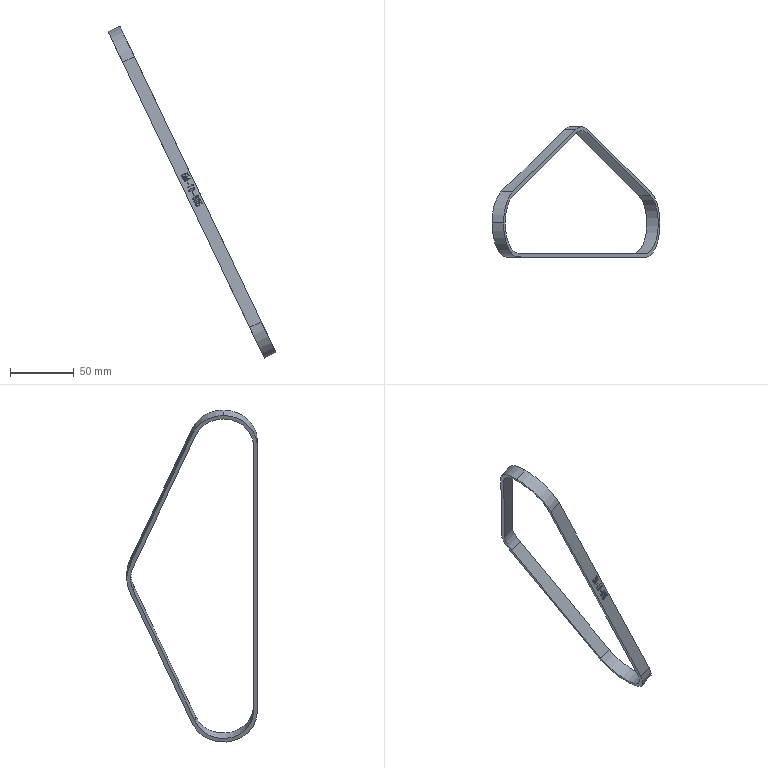Component | SolidWorks | TimingBelt5M-10-625-1 | 1 solid | 183 faces | box 131.26 x 102.19 x 259.67 mm | volume 19104 mm3 | plane 102 | spline 73 | cylinder 8 | commonest cylinder face diameters 47.1 x3 53.1 x3 56.254 x1 50.254 x1
build123d program:
from build123d import *

# Parameters (mm, degrees)
BOSS_EXTRUDE1_DEPTH = 10
SKETCH2_W           = 3.401
SKETCH2_H           = 0.341
CUT_EXTRUDE1_DEPTH  = 1


with BuildPart() as part:
    # Sketch1 → Boss-Extrude1 (new body)
    with BuildSketch(Plane.XY):
        with BuildLine():
            Line((-125.448, 13.156), (-11.068, 62.116))
            ThreePointArc((-11.068, 62.116), (0, 64.386), (11.068, 62.116))
            Line((11.068, 62.116), (125.448, 13.156))
            ThreePointArc((125.448, 13.156), (141.009, -16.584), (115, -37.802))
            Line((115, -37.802), (-115, -37.802))
            ThreePointArc((-115, -37.802), (-141.009, -16.584), (-125.448, 13.156))
        make_face()
        with BuildLine():
            Line((-124.267, 10.398), (-9.888, 59.359))
            ThreePointArc((-9.888, 59.359), (0, 61.386), (9.888, 59.359))
            Line((9.888, 59.359), (124.267, 10.398))
            ThreePointArc((124.267, 10.398), (138.07, -15.982), (115, -34.802))
            Line((115, -34.802), (-115, -34.802))
            ThreePointArc((-115, -34.802), (-138.07, -15.982), (-124.267, 10.398))
        make_face(mode=Mode.SUBTRACT)
    extrude(amount=BOSS_EXTRUDE1_DEPTH)

    # Sketch2 → Cut-Extrude1 (cut)
    # profile 1 of 9: a face of its own
    with BuildSketch(Plane.XZ.offset(37.802)):
        with BuildLine():
            add(Edge.make_bspline(
                [(-15.016, 8.016), (-14.998, 8.018), (-14.966, 8.021), (-14.934, 8.028), (-14.921, 8.031)],
                knots=[0, 0, 0, 0, 1.154, 2, 2, 2, 2], degree=3))
            Line((-14.921, 8.031), (-14.755, 8.039))
            Line((-14.755, 8.039), (-14.446, 8.086))
            Line((-14.446, 8.086), (-14.185, 8.118))
            add(Edge.make_bspline(
                [(-14.185, 8.118), (-14.161, 8.121), (-14.109, 8.13), (-14.061, 8.148), (-14.035, 8.157)],
                knots=[0, 0, 0, 0, 0.9516, 2, 2, 2, 2], degree=3))
            Line((-14.035, 8.157), (-13.917, 8.205))
            add(Edge.make_bspline(
                [(-13.917, 8.205), (-13.905, 8.21), (-13.883, 8.218), (-13.856, 8.23), (-13.836, 8.238), (-13.826, 8.243), (-13.822, 8.244)],
                knots=[0, 0, 0, 0, 1.52, 2.667, 3.508, 4, 4, 4, 4], degree=3))
            Line((-13.822, 8.244), (-13.75, 8.292))
            Line((-13.75, 8.292), (-13.521, 8.062))
            add(Edge.make_bspline(
                [(-13.521, 8.062), (-13.512, 8.051), (-13.497, 8.031), (-13.491, 7.996), (-13.499, 7.971), (-13.507, 7.949), (-13.531, 7.936), (-13.549, 7.936), (-13.56, 7.936)],
                knots=[0, 0, 0, 0, 1.453, 2.543, 3.406, 4.121, 4.875, 6, 6, 6, 6], degree=3))
            Line((-13.56, 7.936), (-15.032, 7.731))
            Line((-15.032, 7.731), (-15.056, 6.124))
            add(Edge.make_bspline(
                [(-15.056, 6.124), (-15.026, 6.16), (-14.971, 6.228), (-14.889, 6.324), (-14.793, 6.406), (-14.695, 6.458), (-14.603, 6.496), (-14.522, 6.515), (-14.432, 6.527), (-14.369, 6.528), (-14.336, 6.528)],
                knots=[0, 0, 0, 0, 1.309, 2.415, 3.508, 4.775, 5.486, 6.257, 7.088, 8, 8, 8, 8], degree=3))
            add(Edge.make_bspline(
                [(-14.336, 6.528), (-14.304, 6.526), (-14.242, 6.522), (-14.157, 6.507), (-14.082, 6.486), (-13.998, 6.442), (-13.898, 6.367), (-13.805, 6.274), (-13.732, 6.184), (-13.678, 6.108), (-13.634, 6.019), (-13.591, 5.925), (-13.553, 5.821), (-13.522, 5.707), (-13.497, 5.582), (-13.47, 5.4), (-13.447, 5.152), (-13.444, 4.949), (-13.442, 4.843)],
                knots=[0, 0, 0, 0, 0.7379, 1.395, 1.969, 2.484, 3.549, 4.783, 5.457, 6.164, 6.905, 7.691, 8.52, 9.412, 10.371, 11.392, 13.598, 16, 16, 16, 16], degree=3))
            add(Edge.make_bspline(
                [(-13.442, 4.843), (-13.444, 4.796), (-13.448, 4.704), (-13.454, 4.572), (-13.465, 4.449), (-13.481, 4.301), (-13.507, 4.131), (-13.553, 3.943), (-13.615, 3.77), (-13.699, 3.614), (-13.793, 3.478), (-13.894, 3.369), (-13.999, 3.29), (-14.11, 3.24), (-14.231, 3.217), (-14.315, 3.214), (-14.36, 3.213)],
                knots=[0, 0, 0, 0, 0.9535, 1.844, 2.674, 3.443, 4.846, 6.127, 7.335, 8.547, 9.683, 10.669, 11.53, 12.306, 13.101, 14, 14, 14, 14], degree=3))
            add(Edge.make_bspline(
                [(-14.36, 3.213), (-14.413, 3.212), (-14.513, 3.21), (-14.655, 3.227), (-14.785, 3.274), (-14.908, 3.346), (-15.023, 3.446), (-15.122, 3.57), (-15.201, 3.703), (-15.258, 3.843), (-15.293, 3.993), (-15.323, 4.157), (-15.343, 4.33), (-15.341, 4.447), (-15.341, 4.503)],
                knots=[0, 0, 0, 0, 1.038, 1.926, 2.77, 3.69, 4.673, 5.718, 6.748, 7.672, 8.626, 9.735, 10.901, 12, 12, 12, 12], degree=3))
            Line((-15.341, 4.503), (-15.332, 4.725))
            Line((-15.332, 4.725), (-15.246, 4.725))
            add(Edge.make_bspline(
                [(-15.246, 4.725), (-15.242, 4.681), (-15.235, 4.593), (-15.219, 4.462), (-15.193, 4.329), (-15.161, 4.195), (-15.12, 4.068), (-15.076, 3.951), (-15.012, 3.845), (-14.935, 3.738), (-14.836, 3.64), (-14.737, 3.572), (-14.647, 3.533), (-14.57, 3.512), (-14.483, 3.501), (-14.423, 3.499), (-14.391, 3.498)],
                knots=[0, 0, 0, 0, 1.118, 2.211, 3.325, 4.532, 5.692, 6.691, 7.681, 8.808, 10, 11.187, 11.809, 12.474, 13.201, 14, 14, 14, 14], degree=3))
            add(Edge.make_bspline(
                [(-14.391, 3.498), (-14.354, 3.498), (-14.279, 3.498), (-14.185, 3.521), (-14.11, 3.556), (-14.053, 3.597), (-13.993, 3.65), (-13.935, 3.717), (-13.878, 3.791), (-13.828, 3.872), (-13.788, 3.96), (-13.746, 4.086), (-13.707, 4.256), (-13.671, 4.476), (-13.653, 4.717), (-13.654, 4.883), (-13.655, 4.97)],
                knots=[0, 0, 0, 0, 0.8494, 1.714, 2.189, 2.722, 3.33, 4.013, 4.74, 5.462, 6.189, 6.935, 8.497, 10.189, 12.026, 14, 14, 14, 14], degree=3))
            add(Edge.make_bspline(
                [(-13.655, 4.97), (-13.658, 5.02), (-13.663, 5.116), (-13.678, 5.254), (-13.693, 5.378), (-13.72, 5.522), (-13.763, 5.688), (-13.824, 5.841), (-13.884, 5.952), (-13.933, 6.026), (-13.989, 6.088), (-14.05, 6.141), (-14.116, 6.184), (-14.185, 6.216), (-14.259, 6.237), (-14.31, 6.241), (-14.336, 6.244)],
                knots=[0, 0, 0, 0, 1.343, 2.566, 3.677, 4.66, 6.478, 8.217, 9.045, 9.823, 10.56, 11.274, 11.966, 12.641, 13.309, 14, 14, 14, 14], degree=3))
            add(Edge.make_bspline(
                [(-14.336, 6.244), (-14.364, 6.243), (-14.419, 6.241), (-14.499, 6.227), (-14.573, 6.202), (-14.661, 6.159), (-14.758, 6.094), (-14.853, 6.007), (-14.926, 5.917), (-14.96, 5.854), (-14.976, 5.824)],
                knots=[0, 0, 0, 0, 0.8403, 1.634, 2.407, 3.158, 4.57, 5.857, 6.993, 8, 8, 8, 8], degree=3))
            Line((-14.976, 5.824), (-15.032, 5.713))
            Line((-15.032, 5.713), (-15.048, 5.611))
            add(Edge.make_bspline(
                [(-15.048, 5.611), (-15.049, 5.597), (-15.05, 5.572), (-15.055, 5.539), (-15.059, 5.519), (-15.061, 5.501), (-15.08, 5.503), (-15.097, 5.52), (-15.128, 5.545), (-15.152, 5.566), (-15.166, 5.579)],
                knots=[0, 0, 0, 0, 1.417, 2.488, 3.243, 3.666, 3.979, 4.774, 6.11, 8, 8, 8, 8], degree=3))
            Line((-15.166, 5.579), (-15.332, 5.713))
            add(Edge.make_bspline(
                [(-15.332, 5.713), (-15.347, 5.726), (-15.369, 5.746), (-15.393, 5.784), (-15.375, 5.824), (-15.359, 5.849), (-15.349, 5.864)],
                knots=[0, 0, 0, 0, 1.303, 2.023, 2.754, 4, 4, 4, 4], degree=3))
            Line((-15.349, 5.864), (-15.261, 5.982))
            Line((-15.261, 5.982), (-15.246, 6.828))
            Line((-15.246, 6.828), (-15.238, 7.438))
            add(Edge.make_bspline(
                [(-15.238, 7.438), (-15.238, 7.46), (-15.238, 7.509), (-15.238, 7.587), (-15.237, 7.675), (-15.238, 7.768), (-15.237, 7.858), (-15.24, 7.934), (-15.241, 7.993), (-15.244, 8.025), (-15.246, 8.039)],
                knots=[0, 0, 0, 0, 0.9041, 1.949, 3.118, 4.412, 5.659, 6.688, 7.452, 8, 8, 8, 8], degree=3))
            Line((-15.246, 8.039), (-15.277, 8.284))
            Line((-15.277, 8.284), (-15.198, 8.316))
            add(Edge.make_bspline(
                [(-15.198, 8.316), (-15.186, 8.286), (-15.167, 8.237), (-15.139, 8.171), (-15.105, 8.122), (-15.078, 8.094), (-15.064, 8.079)],
                knots=[0, 0, 0, 0, 1.379, 2.319, 3.105, 4, 4, 4, 4], degree=3))
            Line((-15.064, 8.079), (-15.016, 8.016))
        make_face()
    # profile 2 of 9: a face of its own
    with BuildSketch(Plane.XZ.offset(37.802)):
        with BuildLine():
            Line((-10.449, 8.347), (-10.267, 8.347))
            Line((-10.267, 8.347), (-10.157, 4.637))
            Line((-10.157, 4.637), (-10.149, 4.289))
            add(Edge.make_bspline(
                [(-10.149, 4.289), (-10.148, 4.25), (-10.148, 4.184), (-10.142, 4.096), (-10.13, 4.023), (-10.115, 3.953), (-10.094, 3.886), (-10.073, 3.829), (-10.052, 3.788), (-10.04, 3.755), (-10.046, 3.723), (-10.055, 3.683), (-10.076, 3.625), (-10.092, 3.58), (-10.101, 3.554)],
                knots=[0, 0, 0, 0, 1.834, 3.115, 4.183, 5.36, 6.502, 7.475, 8.229, 8.746, 9.081, 9.728, 10.706, 12, 12, 12, 12], degree=3))
            Line((-10.101, 3.554), (-10.189, 3.284))
            add(Edge.make_bspline(
                [(-10.189, 3.284), (-10.198, 3.26), (-10.215, 3.216), (-10.239, 3.16), (-10.255, 3.122), (-10.271, 3.097), (-10.287, 3.084), (-10.307, 3.08), (-10.322, 3.093), (-10.328, 3.104), (-10.331, 3.111)],
                knots=[0, 0, 0, 0, 2.257, 3.989, 5.166, 5.812, 6.432, 6.936, 7.389, 8, 8, 8, 8], degree=3))
            add(Edge.make_bspline(
                [(-10.331, 3.111), (-10.335, 3.121), (-10.348, 3.145), (-10.348, 3.196), (-10.348, 3.265), (-10.342, 3.318), (-10.339, 3.348)],
                knots=[0, 0, 0, 0, 0.5334, 1.357, 2.51, 4, 4, 4, 4], degree=3))
            Line((-10.339, 3.348), (-10.354, 3.846))
            Line((-10.354, 3.846), (-10.449, 7.271))
            Line((-10.449, 7.271), (-11.335, 3.253))
            Line((-11.335, 3.253), (-11.486, 3.261))
            Line((-11.486, 3.261), (-12.442, 7.225))
            Line((-12.442, 7.225), (-12.506, 3.807))
            Line((-12.506, 3.807), (-12.522, 3.316))
            add(Edge.make_bspline(
                [(-12.522, 3.316), (-12.522, 3.28), (-12.523, 3.217), (-12.534, 3.143), (-12.545, 3.098), (-12.554, 3.077), (-12.564, 3.062), (-12.573, 3.063), (-12.577, 3.063)],
                knots=[0, 0, 0, 0, 2.359, 4.22, 4.917, 5.428, 5.74, 6, 6, 6, 6], degree=3))
            add(Edge.make_bspline(
                [(-12.577, 3.063), (-12.583, 3.064), (-12.594, 3.066), (-12.616, 3.076), (-12.632, 3.112), (-12.646, 3.153), (-12.659, 3.192), (-12.665, 3.217), (-12.671, 3.233), (-12.672, 3.242), (-12.672, 3.245)],
                knots=[0, 0, 0, 0, 0.6183, 1.294, 2.516, 4.811, 6.123, 7.066, 7.695, 8, 8, 8, 8], degree=3))
            Line((-12.672, 3.245), (-12.815, 3.601))
            add(Edge.make_bspline(
                [(-12.815, 3.601), (-12.819, 3.619), (-12.827, 3.654), (-12.825, 3.709), (-12.81, 3.768), (-12.788, 3.829), (-12.765, 3.885), (-12.749, 3.927), (-12.74, 3.958), (-12.736, 3.99), (-12.731, 4.031), (-12.728, 4.079), (-12.725, 4.128), (-12.721, 4.17), (-12.72, 4.201), (-12.717, 4.223), (-12.715, 4.241), (-12.714, 4.264), (-12.713, 4.296), (-12.71, 4.338), (-12.71, 4.389), (-12.707, 4.45), (-12.706, 4.521), (-12.705, 4.571), (-12.704, 4.598)],
                knots=[0, 0, 0, 0, 1.188, 2.333, 3.586, 5.123, 6.574, 7.524, 7.999, 8.693, 9.59, 10.712, 11.859, 12.753, 13.442, 13.903, 14.184, 14.668, 15.356, 16.273, 17.393, 18.717, 20.244, 22, 22, 22, 22], degree=3))
            Line((-12.704, 4.598), (-12.649, 8.347))
            Line((-12.649, 8.347), (-12.459, 8.347))
            Line((-12.459, 8.347), (-11.423, 3.87))
            Line((-11.423, 3.87), (-10.449, 8.347))
        make_face()
    # profile 3 of 9: a face of its own
    with BuildSketch(Plane.XZ.offset(37.802)):
        with Locations((-7.963, 5.155)):
            Rectangle(SKETCH2_W, SKETCH2_H)
    # profile 4 of 9: a face of its own
    with BuildSketch(Plane.XZ.offset(37.802)):
        with BuildLine():
            Line((-4.557, 8.3), (-4.471, 8.3))
            Line((-4.471, 8.3), (-4.479, 4.099))
            add(Edge.make_bspline(
                [(-4.479, 4.099), (-4.48, 4.061), (-4.482, 3.988), (-4.482, 3.884), (-4.485, 3.79), (-4.486, 3.706), (-4.488, 3.631), (-4.491, 3.566), (-4.491, 3.511), (-4.496, 3.425), (-4.503, 3.306), (-4.518, 3.184), (-4.53, 3.097), (-4.543, 3.057), (-4.558, 3.026), (-4.574, 3.03), (-4.581, 3.031)],
                knots=[0, 0, 0, 0, 1.45, 2.781, 3.977, 5.054, 6.011, 6.834, 7.536, 8.12, 10.143, 12.069, 12.873, 13.44, 13.76, 14, 14, 14, 14], degree=3))
            add(Edge.make_bspline(
                [(-4.581, 3.031), (-4.582, 3.032), (-4.589, 3.037), (-4.605, 3.048), (-4.624, 3.077), (-4.632, 3.102), (-4.637, 3.118)],
                knots=[0, 0, 0, 0, 0.2213, 0.9471, 2.151, 4, 4, 4, 4], degree=3))
            Line((-4.637, 3.118), (-4.676, 3.221))
            Line((-4.676, 3.221), (-4.764, 3.506))
            add(Edge.make_bspline(
                [(-4.764, 3.506), (-4.774, 3.533), (-4.793, 3.579), (-4.811, 3.641), (-4.825, 3.68), (-4.829, 3.712), (-4.811, 3.742), (-4.798, 3.787), (-4.777, 3.846), (-4.758, 3.915), (-4.741, 3.99), (-4.726, 4.071), (-4.717, 4.162), (-4.713, 4.248), (-4.709, 4.332), (-4.709, 4.413), (-4.707, 4.508), (-4.707, 4.577), (-4.707, 4.613)],
                knots=[0, 0, 0, 0, 1.22, 2.126, 2.712, 2.994, 3.44, 4.126, 5.031, 6.063, 7.167, 8.277, 9.542, 11.034, 11.961, 13.087, 14.444, 16, 16, 16, 16], degree=3))
            Line((-4.707, 4.613), (-4.7, 7.714))
            Line((-4.7, 7.714), (-5.112, 7.358))
            Line((-5.112, 7.358), (-5.143, 7.493))
            add(Edge.make_bspline(
                [(-5.143, 7.493), (-5.11, 7.527), (-5.047, 7.592), (-4.964, 7.685), (-4.895, 7.766), (-4.823, 7.861), (-4.743, 7.979), (-4.683, 8.075), (-4.652, 8.126)],
                knots=[0, 0, 0, 0, 1.077, 2.019, 2.808, 3.458, 4.679, 6, 6, 6, 6], degree=3))
            Line((-4.652, 8.126), (-4.557, 8.3))
        make_face()
    # profile 5 of 9: a face of its own
    with BuildSketch(Plane.XZ.offset(37.802)):
        with BuildLine():
            add(Edge.make_bspline(
                [(-2.673, 5.832), (-2.669, 5.908), (-2.661, 6.063), (-2.64, 6.301), (-2.609, 6.55), (-2.572, 6.805), (-2.522, 7.057), (-2.458, 7.297), (-2.375, 7.518), (-2.293, 7.688), (-2.224, 7.813), (-2.173, 7.896), (-2.125, 7.971), (-2.078, 8.036), (-2.032, 8.091), (-1.989, 8.139), (-1.945, 8.177), (-1.891, 8.214), (-1.825, 8.247), (-1.749, 8.276), (-1.675, 8.292), (-1.627, 8.292), (-1.604, 8.292)],
                knots=[0, 0, 0, 0, 1.583, 3.244, 4.984, 6.805, 8.617, 10.34, 11.975, 13.538, 14.275, 14.951, 15.564, 16.129, 16.627, 17.071, 17.469, 17.815, 18.438, 19.003, 19.519, 20, 20, 20, 20], degree=3))
            add(Edge.make_bspline(
                [(-1.604, 8.292), (-1.582, 8.288), (-1.535, 8.28), (-1.466, 8.25), (-1.393, 8.209), (-1.315, 8.157), (-1.237, 8.087), (-1.165, 7.993), (-1.098, 7.88), (-1.015, 7.7), (-0.9231, 7.455), (-0.8511, 7.199), (-0.8044, 6.985), (-0.7739, 6.814), (-0.7496, 6.633), (-0.7235, 6.378), (-0.7003, 6.052), (-0.6966, 5.789), (-0.6947, 5.658)],
                knots=[0, 0, 0, 0, 0.3637, 0.7682, 1.217, 1.725, 2.291, 2.915, 3.632, 4.434, 6.138, 7.867, 8.757, 9.699, 10.686, 11.727, 13.859, 16, 16, 16, 16], degree=3))
            add(Edge.make_bspline(
                [(-0.6947, 5.658), (-0.7019, 5.552), (-0.7166, 5.335), (-0.7517, 5.003), (-0.8095, 4.657), (-0.8823, 4.366), (-0.9528, 4.135), (-1.012, 3.967), (-1.079, 3.81), (-1.151, 3.662), (-1.225, 3.531), (-1.302, 3.421), (-1.383, 3.337), (-1.466, 3.276), (-1.547, 3.235), (-1.625, 3.208), (-1.699, 3.194), (-1.747, 3.196), (-1.771, 3.198)],
                knots=[0, 0, 0, 0, 1.76, 3.618, 5.557, 7.587, 8.607, 9.588, 10.541, 11.46, 12.308, 13.044, 13.688, 14.251, 14.754, 15.2, 15.616, 16, 16, 16, 16], degree=3))
            add(Edge.make_bspline(
                [(-1.771, 3.198), (-1.793, 3.201), (-1.839, 3.207), (-1.909, 3.235), (-1.982, 3.277), (-2.06, 3.333), (-2.139, 3.41), (-2.214, 3.509), (-2.287, 3.631), (-2.355, 3.774), (-2.42, 3.934), (-2.477, 4.106), (-2.529, 4.286), (-2.571, 4.475), (-2.606, 4.666), (-2.633, 4.854), (-2.652, 5.036), (-2.662, 5.212), (-2.666, 5.38), (-2.67, 5.54), (-2.672, 5.689), (-2.673, 5.786), (-2.673, 5.832)],
                knots=[0, 0, 0, 0, 0.4512, 0.9506, 1.515, 2.163, 2.892, 3.734, 4.688, 5.773, 6.954, 8.176, 9.446, 10.772, 12.102, 13.384, 14.62, 15.819, 16.962, 18.041, 19.056, 20, 20, 20, 20], degree=3))
        make_face()
        with BuildLine():
            add(Edge.make_bspline(
                [(-2.467, 5.816), (-2.468, 5.778), (-2.469, 5.697), (-2.471, 5.569), (-2.468, 5.427), (-2.462, 5.216), (-2.443, 4.941), (-2.392, 4.611), (-2.32, 4.291), (-2.241, 4.041), (-2.167, 3.862), (-2.111, 3.751), (-2.051, 3.662), (-1.989, 3.594), (-1.926, 3.545), (-1.867, 3.511), (-1.811, 3.487), (-1.773, 3.484), (-1.755, 3.482)],
                knots=[0, 0, 0, 0, 0.7057, 1.499, 2.386, 3.361, 5.418, 7.515, 9.574, 11.515, 12.399, 13.17, 13.83, 14.396, 14.883, 15.304, 15.67, 16, 16, 16, 16], degree=3))
            add(Edge.make_bspline(
                [(-1.755, 3.482), (-1.739, 3.483), (-1.704, 3.483), (-1.648, 3.496), (-1.59, 3.524), (-1.526, 3.561), (-1.459, 3.618), (-1.394, 3.695), (-1.33, 3.794), (-1.266, 3.912), (-1.205, 4.042), (-1.151, 4.18), (-1.104, 4.323), (-1.053, 4.523), (-1.001, 4.781), (-0.9537, 5.098), (-0.9225, 5.409), (-0.9095, 5.664), (-0.9059, 5.865), (-0.9089, 6.025), (-0.9146, 6.197), (-0.921, 6.316), (-0.9244, 6.377)],
                knots=[0, 0, 0, 0, 0.3081, 0.6619, 1.055, 1.515, 2.051, 2.68, 3.41, 4.262, 5.184, 6.105, 7.046, 8, 9.968, 11.998, 13.994, 15.843, 16.773, 17.77, 18.848, 20, 20, 20, 20], degree=3))
            add(Edge.make_bspline(
                [(-0.9244, 6.377), (-0.9301, 6.435), (-0.941, 6.546), (-0.9603, 6.707), (-0.9842, 6.857), (-1.018, 7.041), (-1.072, 7.262), (-1.147, 7.473), (-1.212, 7.632), (-1.268, 7.732), (-1.324, 7.818), (-1.387, 7.883), (-1.448, 7.934), (-1.506, 7.972), (-1.56, 7.999), (-1.596, 8.005), (-1.612, 8.007)],
                knots=[0, 0, 0, 0, 1.303, 2.529, 3.662, 4.721, 6.756, 8.792, 9.76, 10.624, 11.385, 12.064, 12.659, 13.175, 13.621, 14, 14, 14, 14], degree=3))
            add(Edge.make_bspline(
                [(-1.612, 8.007), (-1.63, 8.006), (-1.668, 8.003), (-1.726, 7.986), (-1.788, 7.958), (-1.856, 7.919), (-1.926, 7.857), (-1.997, 7.767), (-2.071, 7.647), (-2.147, 7.499), (-2.221, 7.324), (-2.283, 7.125), (-2.337, 6.903), (-2.378, 6.666), (-2.41, 6.429), (-2.436, 6.206), (-2.456, 6.004), (-2.463, 5.876), (-2.467, 5.816)],
                knots=[0, 0, 0, 0, 0.3474, 0.73, 1.157, 1.645, 2.22, 2.946, 3.85, 4.924, 6.146, 7.478, 8.938, 10.524, 12.101, 13.544, 14.841, 16, 16, 16, 16], degree=3))
        make_face(mode=Mode.SUBTRACT)
    # profile 6 of 9: a face of its own
    with BuildSketch(Plane.XZ.offset(37.802)):
        with Locations((1.713, 5.155)):
            Rectangle(SKETCH2_W, SKETCH2_H)
    # profile 7 of 9: a face of its own
    with BuildSketch(Plane.XZ.offset(37.802)):
        with BuildLine():
            Line((6.019, 6.797), (5.909, 6.797))
            add(Edge.make_bspline(
                [(5.909, 6.797), (5.902, 6.844), (5.887, 6.937), (5.873, 7.08), (5.856, 7.228), (5.828, 7.385), (5.783, 7.548), (5.719, 7.678), (5.659, 7.775), (5.608, 7.84), (5.549, 7.895), (5.487, 7.941), (5.419, 7.976), (5.348, 8.002), (5.273, 8.013), (5.197, 8.012), (5.122, 8.004), (5.053, 7.986), (4.991, 7.961), (4.933, 7.929), (4.88, 7.882), (4.824, 7.824), (4.769, 7.747), (4.711, 7.657), (4.654, 7.552), (4.605, 7.432), (4.56, 7.299), (4.509, 7.103), (4.461, 6.839), (4.432, 6.569), (4.418, 6.358), (4.412, 6.216), (4.406, 6.093), (4.406, 6.017), (4.406, 5.982)],
                knots=[0, 0, 0, 0, 1.173, 2.32, 3.517, 4.833, 6.232, 7.655, 8.357, 9.032, 9.677, 10.315, 10.933, 11.542, 12.153, 12.786, 13.414, 13.988, 14.535, 15.054, 15.605, 16.263, 17.03, 17.918, 18.896, 19.957, 21.1, 22.329, 24.933, 27.662, 28.978, 30.14, 31.147, 32, 32, 32, 32], degree=3))
            Line((4.406, 5.982), (4.399, 5.674))
            add(Edge.make_bspline(
                [(4.399, 5.674), (4.418, 5.729), (4.454, 5.829), (4.508, 5.967), (4.569, 6.083), (4.641, 6.191), (4.734, 6.291), (4.828, 6.364), (4.918, 6.414), (4.997, 6.443), (5.086, 6.463), (5.149, 6.469), (5.182, 6.472)],
                knots=[0, 0, 0, 0, 1.464, 2.646, 3.694, 4.755, 5.874, 7.079, 7.725, 8.423, 9.174, 10, 10, 10, 10], degree=3))
            add(Edge.make_bspline(
                [(5.182, 6.472), (5.229, 6.47), (5.319, 6.467), (5.45, 6.428), (5.571, 6.36), (5.665, 6.276), (5.741, 6.194), (5.797, 6.118), (5.851, 6.033), (5.921, 5.905), (5.996, 5.73), (6.051, 5.544), (6.079, 5.386), (6.098, 5.259), (6.107, 5.123), (6.113, 4.933), (6.11, 4.696), (6.097, 4.507), (6.091, 4.415)],
                knots=[0, 0, 0, 0, 0.9091, 1.729, 2.577, 3.565, 4.121, 4.72, 5.36, 6.06, 7.513, 8.994, 9.771, 10.587, 11.458, 12.38, 14.23, 16, 16, 16, 16], degree=3))
            add(Edge.make_bspline(
                [(6.091, 4.415), (6.084, 4.368), (6.068, 4.269), (6.036, 4.116), (5.996, 3.954), (5.95, 3.788), (5.897, 3.63), (5.827, 3.496), (5.742, 3.391), (5.645, 3.318), (5.548, 3.271), (5.461, 3.234), (5.386, 3.207), (5.338, 3.201), (5.316, 3.198)],
                knots=[0, 0, 0, 0, 1.11, 2.303, 3.588, 4.949, 6.256, 7.397, 8.411, 9.334, 10.174, 10.886, 11.5, 12, 12, 12, 12], degree=3))
            add(Edge.make_bspline(
                [(5.316, 3.198), (5.277, 3.194), (5.198, 3.188), (5.099, 3.206), (5.019, 3.234), (4.954, 3.267), (4.882, 3.307), (4.808, 3.36), (4.732, 3.421), (4.664, 3.497), (4.601, 3.581), (4.529, 3.709), (4.453, 3.878), (4.382, 4.054), (4.337, 4.21), (4.306, 4.349), (4.277, 4.511), (4.252, 4.688), (4.23, 4.862), (4.211, 5.018), (4.195, 5.148), (4.181, 5.287), (4.171, 5.44), (4.168, 5.621), (4.171, 5.812), (4.175, 5.944), (4.177, 6.014)],
                knots=[0, 0, 0, 0, 0.8482, 1.691, 2.145, 2.659, 3.249, 3.913, 4.622, 5.34, 6.091, 6.877, 8.487, 10.078, 10.944, 11.968, 13.145, 14.476, 15.796, 16.92, 17.858, 18.609, 19.904, 21.163, 22.497, 24, 24, 24, 24], degree=3))
            add(Edge.make_bspline(
                [(4.177, 6.014), (4.179, 6.07), (4.181, 6.175), (4.187, 6.323), (4.193, 6.45), (4.207, 6.596), (4.229, 6.775), (4.263, 6.995), (4.303, 7.215), (4.348, 7.391), (4.39, 7.527), (4.43, 7.63), (4.48, 7.736), (4.534, 7.845), (4.597, 7.949), (4.665, 8.042), (4.739, 8.121), (4.818, 8.188), (4.908, 8.238), (5.007, 8.274), (5.119, 8.292), (5.196, 8.292), (5.237, 8.292)],
                knots=[0, 0, 0, 0, 1.212, 2.28, 3.204, 3.978, 5.462, 7.117, 8.789, 10.309, 11.065, 11.864, 12.713, 13.607, 14.507, 15.33, 16.109, 16.844, 17.564, 18.32, 19.127, 20, 20, 20, 20], degree=3))
            add(Edge.make_bspline(
                [(5.237, 8.292), (5.277, 8.289), (5.355, 8.282), (5.461, 8.253), (5.552, 8.215), (5.625, 8.16), (5.682, 8.1), (5.734, 8.046), (5.775, 7.99), (5.811, 7.936), (5.841, 7.876), (5.871, 7.808), (5.898, 7.727), (5.925, 7.64), (5.95, 7.551), (5.971, 7.469), (5.987, 7.397), (6.004, 7.31), (6.018, 7.195), (6.019, 7.101), (6.019, 7.05)],
                knots=[0, 0, 0, 0, 1.358, 2.566, 3.646, 4.63, 5.547, 6.392, 7.141, 7.836, 8.549, 9.369, 10.304, 11.363, 12.414, 13.352, 14.176, 14.876, 16.3, 18, 18, 18, 18], degree=3))
            Line((6.019, 7.05), (6.019, 6.797))
        make_face()
        with BuildLine():
            add(Edge.make_bspline(
                [(4.501, 4.843), (4.503, 4.773), (4.508, 4.628), (4.537, 4.409), (4.589, 4.187), (4.65, 4.005), (4.711, 3.865), (4.766, 3.771), (4.825, 3.686), (4.893, 3.612), (4.968, 3.55), (5.054, 3.51), (5.147, 3.487), (5.211, 3.489), (5.245, 3.491)],
                knots=[0, 0, 0, 0, 1.489, 3.055, 4.666, 6.307, 7.113, 7.875, 8.604, 9.311, 9.987, 10.645, 11.298, 12, 12, 12, 12], degree=3))
            add(Edge.make_bspline(
                [(5.245, 3.491), (5.274, 3.493), (5.331, 3.499), (5.415, 3.529), (5.495, 3.574), (5.571, 3.635), (5.639, 3.708), (5.7, 3.789), (5.75, 3.877), (5.801, 4.007), (5.849, 4.186), (5.875, 4.416), (5.891, 4.656), (5.904, 4.904), (5.901, 5.161), (5.87, 5.333), (5.854, 5.421)],
                knots=[0, 0, 0, 0, 0.5424, 1.087, 1.661, 2.274, 2.914, 3.54, 4.173, 4.817, 6.174, 7.637, 9.172, 10.719, 12.317, 14, 14, 14, 14], degree=3))
            add(Edge.make_bspline(
                [(5.854, 5.421), (5.833, 5.493), (5.79, 5.636), (5.709, 5.803), (5.633, 5.923), (5.577, 6), (5.515, 6.06), (5.453, 6.108), (5.388, 6.142), (5.324, 6.168), (5.257, 6.18), (5.212, 6.18), (5.19, 6.18)],
                knots=[0, 0, 0, 0, 2.077, 4.127, 5.096, 5.974, 6.759, 7.476, 8.137, 8.771, 9.385, 10, 10, 10, 10], degree=3))
            add(Edge.make_bspline(
                [(5.19, 6.18), (5.163, 6.176), (5.108, 6.168), (5.029, 6.139), (4.954, 6.097), (4.862, 6.024), (4.762, 5.923), (4.684, 5.805), (4.639, 5.702), (4.606, 5.614), (4.577, 5.512), (4.55, 5.398), (4.528, 5.273), (4.512, 5.138), (4.503, 4.994), (4.501, 4.894), (4.501, 4.843)],
                knots=[0, 0, 0, 0, 0.7035, 1.417, 2.139, 2.91, 4.405, 5.781, 6.485, 7.297, 8.194, 9.202, 10.291, 11.452, 12.687, 14, 14, 14, 14], degree=3))
        make_face(mode=Mode.SUBTRACT)
    # profile 8 of 9: a face of its own
    with BuildSketch(Plane.XZ.offset(37.802)):
        with BuildLine():
            Line((7.122, 6.259), (7.003, 6.259))
            add(Edge.make_bspline(
                [(7.003, 6.259), (7, 6.297), (6.996, 6.369), (6.991, 6.472), (6.989, 6.565), (6.987, 6.678), (6.99, 6.82), (6.998, 6.935), (7.003, 6.995)],
                knots=[0, 0, 0, 0, 0.9275, 1.768, 2.523, 3.191, 4.527, 6, 6, 6, 6], degree=3))
            add(Edge.make_bspline(
                [(7.003, 6.995), (7.006, 7.039), (7.012, 7.126), (7.027, 7.25), (7.046, 7.365), (7.069, 7.473), (7.101, 7.579), (7.147, 7.686), (7.204, 7.797), (7.271, 7.908), (7.344, 8.013), (7.427, 8.098), (7.513, 8.163), (7.605, 8.202), (7.693, 8.226), (7.774, 8.245), (7.846, 8.258), (7.892, 8.26), (7.913, 8.261)],
                knots=[0, 0, 0, 0, 1.239, 2.395, 3.471, 4.469, 5.466, 6.534, 7.677, 8.916, 10.134, 11.221, 12.198, 13.11, 13.967, 14.734, 15.403, 16, 16, 16, 16], degree=3))
            add(Edge.make_bspline(
                [(7.913, 8.261), (7.941, 8.258), (7.995, 8.254), (8.075, 8.236), (8.152, 8.209), (8.25, 8.162), (8.366, 8.087), (8.464, 7.989), (8.531, 7.899), (8.579, 7.823), (8.622, 7.738), (8.675, 7.614), (8.73, 7.45), (8.77, 7.242), (8.796, 7.027), (8.808, 6.806), (8.81, 6.588), (8.797, 6.446), (8.791, 6.377)],
                knots=[0, 0, 0, 0, 0.5708, 1.128, 1.695, 2.261, 3.397, 4.528, 5.118, 5.731, 6.395, 7.093, 8.529, 9.987, 11.474, 13.035, 14.568, 16, 16, 16, 16], degree=3))
            add(Edge.make_bspline(
                [(8.791, 6.377), (8.779, 6.307), (8.753, 6.164), (8.699, 5.993), (8.648, 5.862), (8.606, 5.775), (8.56, 5.698), (8.495, 5.606), (8.395, 5.502), (8.302, 5.433), (8.253, 5.396)],
                knots=[0, 0, 0, 0, 1.491, 3.004, 3.73, 4.398, 5.021, 5.591, 6.734, 8, 8, 8, 8], degree=3))
            Line((8.253, 5.396), (7.865, 5.151))
            add(Edge.make_bspline(
                [(7.865, 5.151), (7.816, 5.118), (7.722, 5.054), (7.597, 4.95), (7.492, 4.841), (7.413, 4.72), (7.351, 4.595), (7.296, 4.47), (7.255, 4.332), (7.225, 4.208), (7.205, 4.104), (7.195, 4.032), (7.187, 3.968), (7.186, 3.928), (7.186, 3.909)],
                knots=[0, 0, 0, 0, 1.454, 2.756, 3.954, 5.133, 6.264, 7.337, 8.453, 9.763, 10.431, 11.027, 11.543, 12, 12, 12, 12], degree=3))
            Line((7.186, 3.909), (7.169, 3.577))
            Line((7.169, 3.577), (8.585, 3.624))
            add(Edge.make_bspline(
                [(8.585, 3.624), (8.603, 3.625), (8.635, 3.627), (8.666, 3.66), (8.672, 3.701), (8.685, 3.752), (8.694, 3.823), (8.7, 3.878), (8.704, 3.909)],
                knots=[0, 0, 0, 0, 0.9259, 1.626, 2.181, 3.087, 4.358, 6, 6, 6, 6], degree=3))
            Line((8.704, 3.909), (8.736, 4.598))
            Line((8.736, 4.598), (8.846, 4.598))
            Line((8.846, 4.598), (8.886, 3.554))
            add(Edge.make_bspline(
                [(8.886, 3.554), (8.887, 3.534), (8.89, 3.498), (8.891, 3.451), (8.891, 3.418), (8.89, 3.392), (8.882, 3.369), (8.874, 3.342), (8.843, 3.327), (8.799, 3.322), (8.732, 3.315), (8.679, 3.316), (8.648, 3.316)],
                knots=[0, 0, 0, 0, 1.385, 2.422, 3.194, 3.62, 4.201, 4.878, 5.403, 6.404, 7.926, 10, 10, 10, 10], degree=3))
            Line((8.648, 3.316), (7.074, 3.276))
            add(Edge.make_bspline(
                [(7.074, 3.276), (7.055, 3.276), (7.017, 3.276), (6.979, 3.314), (6.963, 3.359), (6.954, 3.413), (6.949, 3.485), (6.946, 3.608), (6.952, 3.784), (6.964, 3.928), (6.971, 4.004)],
                knots=[0, 0, 0, 0, 0.5564, 1.097, 1.476, 2.013, 2.731, 3.636, 5.715, 8, 8, 8, 8], degree=3))
            add(Edge.make_bspline(
                [(6.971, 4.004), (6.977, 4.048), (6.988, 4.133), (7.011, 4.256), (7.035, 4.37), (7.062, 4.475), (7.091, 4.57), (7.123, 4.656), (7.156, 4.734), (7.206, 4.822), (7.269, 4.918), (7.341, 5.021), (7.41, 5.109), (7.501, 5.206), (7.623, 5.311), (7.726, 5.388), (7.779, 5.428)],
                knots=[0, 0, 0, 0, 1.103, 2.126, 3.085, 3.983, 4.803, 5.556, 6.253, 6.893, 8.055, 9.095, 10.01, 10.818, 12.366, 14, 14, 14, 14], degree=3))
            Line((7.779, 5.428), (8.103, 5.634))
            add(Edge.make_bspline(
                [(8.103, 5.634), (8.129, 5.651), (8.179, 5.685), (8.248, 5.737), (8.307, 5.792), (8.357, 5.851), (8.403, 5.92), (8.441, 6.005), (8.481, 6.105), (8.527, 6.262), (8.575, 6.468), (8.593, 6.723), (8.583, 6.981), (8.553, 7.152), (8.538, 7.24)],
                knots=[0, 0, 0, 0, 0.6356, 1.22, 1.766, 2.268, 2.802, 3.436, 4.161, 5.002, 6.753, 8.461, 10.189, 12, 12, 12, 12], degree=3))
            add(Edge.make_bspline(
                [(8.538, 7.24), (8.526, 7.284), (8.504, 7.372), (8.461, 7.497), (8.406, 7.611), (8.347, 7.718), (8.273, 7.812), (8.175, 7.879), (8.058, 7.924), (7.973, 7.932), (7.929, 7.936)],
                knots=[0, 0, 0, 0, 1.101, 2.148, 3.157, 4.125, 5.059, 5.969, 6.936, 8, 8, 8, 8], degree=3))
            add(Edge.make_bspline(
                [(7.929, 7.936), (7.905, 7.936), (7.858, 7.937), (7.789, 7.926), (7.721, 7.904), (7.632, 7.864), (7.529, 7.789), (7.42, 7.676), (7.331, 7.538), (7.262, 7.378), (7.211, 7.196), (7.169, 6.992), (7.141, 6.764), (7.133, 6.604), (7.129, 6.52)],
                knots=[0, 0, 0, 0, 0.4693, 0.9361, 1.404, 1.894, 2.887, 3.927, 5.012, 6.157, 7.397, 8.794, 10.323, 12, 12, 12, 12], degree=3))
            Line((7.129, 6.52), (7.122, 6.259))
        make_face()
    # profile 9 of 9: a face of its own
    with BuildSketch(Plane.XZ.offset(37.802)):
        with BuildLine():
            add(Edge.make_bspline(
                [(10.186, 8.016), (10.204, 8.018), (10.236, 8.021), (10.267, 8.028), (10.281, 8.031)],
                knots=[0, 0, 0, 0, 1.154, 2, 2, 2, 2], degree=3))
            Line((10.281, 8.031), (10.447, 8.039))
            Line((10.447, 8.039), (10.755, 8.086))
            Line((10.755, 8.086), (11.017, 8.118))
            add(Edge.make_bspline(
                [(11.017, 8.118), (11.041, 8.121), (11.092, 8.13), (11.141, 8.148), (11.167, 8.157)],
                knots=[0, 0, 0, 0, 0.9516, 2, 2, 2, 2], degree=3))
            Line((11.167, 8.157), (11.285, 8.205))
            add(Edge.make_bspline(
                [(11.285, 8.205), (11.297, 8.21), (11.319, 8.218), (11.346, 8.23), (11.366, 8.238), (11.376, 8.243), (11.38, 8.244)],
                knots=[0, 0, 0, 0, 1.52, 2.667, 3.508, 4, 4, 4, 4], degree=3))
            Line((11.38, 8.244), (11.451, 8.292))
            Line((11.451, 8.292), (11.681, 8.062))
            add(Edge.make_bspline(
                [(11.681, 8.062), (11.69, 8.051), (11.705, 8.031), (11.71, 7.996), (11.703, 7.971), (11.695, 7.949), (11.671, 7.936), (11.652, 7.936), (11.641, 7.936)],
                knots=[0, 0, 0, 0, 1.453, 2.543, 3.406, 4.121, 4.875, 6, 6, 6, 6], degree=3))
            Line((11.641, 7.936), (10.169, 7.731))
            Line((10.169, 7.731), (10.146, 6.124))
            add(Edge.make_bspline(
                [(10.146, 6.124), (10.176, 6.16), (10.231, 6.228), (10.313, 6.324), (10.409, 6.406), (10.507, 6.458), (10.599, 6.496), (10.68, 6.515), (10.77, 6.527), (10.833, 6.528), (10.865, 6.528)],
                knots=[0, 0, 0, 0, 1.309, 2.415, 3.508, 4.775, 5.486, 6.257, 7.088, 8, 8, 8, 8], degree=3))
            add(Edge.make_bspline(
                [(10.865, 6.528), (10.898, 6.526), (10.959, 6.522), (11.045, 6.507), (11.119, 6.486), (11.204, 6.442), (11.303, 6.367), (11.397, 6.274), (11.47, 6.184), (11.523, 6.108), (11.568, 6.019), (11.61, 5.925), (11.648, 5.821), (11.68, 5.707), (11.705, 5.582), (11.732, 5.4), (11.755, 5.152), (11.758, 4.949), (11.76, 4.843)],
                knots=[0, 0, 0, 0, 0.7379, 1.395, 1.969, 2.484, 3.549, 4.783, 5.457, 6.164, 6.905, 7.691, 8.52, 9.412, 10.371, 11.392, 13.598, 16, 16, 16, 16], degree=3))
            add(Edge.make_bspline(
                [(11.76, 4.843), (11.758, 4.796), (11.754, 4.704), (11.748, 4.572), (11.737, 4.449), (11.72, 4.301), (11.695, 4.131), (11.649, 3.943), (11.587, 3.77), (11.503, 3.614), (11.409, 3.478), (11.308, 3.369), (11.203, 3.29), (11.092, 3.24), (10.971, 3.217), (10.887, 3.214), (10.842, 3.213)],
                knots=[0, 0, 0, 0, 0.9535, 1.844, 2.674, 3.443, 4.846, 6.127, 7.335, 8.547, 9.683, 10.669, 11.53, 12.306, 13.101, 14, 14, 14, 14], degree=3))
            add(Edge.make_bspline(
                [(10.842, 3.213), (10.789, 3.212), (10.689, 3.21), (10.547, 3.227), (10.417, 3.274), (10.294, 3.346), (10.179, 3.446), (10.08, 3.57), (10.001, 3.703), (9.944, 3.843), (9.909, 3.993), (9.879, 4.157), (9.859, 4.33), (9.86, 4.447), (9.861, 4.503)],
                knots=[0, 0, 0, 0, 1.038, 1.926, 2.77, 3.69, 4.673, 5.718, 6.748, 7.672, 8.626, 9.735, 10.901, 12, 12, 12, 12], degree=3))
            Line((9.861, 4.503), (9.869, 4.725))
            Line((9.869, 4.725), (9.956, 4.725))
            add(Edge.make_bspline(
                [(9.956, 4.725), (9.96, 4.681), (9.967, 4.593), (9.983, 4.462), (10.009, 4.329), (10.04, 4.195), (10.082, 4.068), (10.126, 3.951), (10.19, 3.845), (10.267, 3.738), (10.366, 3.64), (10.464, 3.572), (10.555, 3.533), (10.632, 3.512), (10.718, 3.501), (10.779, 3.499), (10.81, 3.498)],
                knots=[0, 0, 0, 0, 1.118, 2.211, 3.325, 4.532, 5.692, 6.691, 7.681, 8.808, 10, 11.187, 11.809, 12.474, 13.201, 14, 14, 14, 14], degree=3))
            add(Edge.make_bspline(
                [(10.81, 3.498), (10.848, 3.498), (10.923, 3.498), (11.017, 3.521), (11.091, 3.556), (11.149, 3.597), (11.209, 3.65), (11.267, 3.717), (11.324, 3.791), (11.374, 3.872), (11.414, 3.96), (11.456, 4.086), (11.495, 4.256), (11.53, 4.476), (11.549, 4.717), (11.547, 4.883), (11.546, 4.97)],
                knots=[0, 0, 0, 0, 0.8494, 1.714, 2.189, 2.722, 3.33, 4.013, 4.74, 5.462, 6.189, 6.935, 8.497, 10.189, 12.026, 14, 14, 14, 14], degree=3))
            add(Edge.make_bspline(
                [(11.546, 4.97), (11.544, 5.02), (11.539, 5.116), (11.524, 5.254), (11.508, 5.378), (11.482, 5.522), (11.439, 5.688), (11.377, 5.841), (11.318, 5.952), (11.269, 6.026), (11.213, 6.088), (11.152, 6.141), (11.086, 6.184), (11.016, 6.216), (10.942, 6.237), (10.891, 6.241), (10.865, 6.244)],
                knots=[0, 0, 0, 0, 1.343, 2.566, 3.677, 4.66, 6.478, 8.217, 9.045, 9.823, 10.56, 11.274, 11.966, 12.641, 13.309, 14, 14, 14, 14], degree=3))
            add(Edge.make_bspline(
                [(10.865, 6.244), (10.837, 6.243), (10.783, 6.241), (10.703, 6.227), (10.629, 6.202), (10.54, 6.159), (10.443, 6.094), (10.349, 6.007), (10.275, 5.917), (10.242, 5.854), (10.226, 5.824)],
                knots=[0, 0, 0, 0, 0.8403, 1.634, 2.407, 3.158, 4.57, 5.857, 6.993, 8, 8, 8, 8], degree=3))
            Line((10.226, 5.824), (10.169, 5.713))
            Line((10.169, 5.713), (10.154, 5.611))
            add(Edge.make_bspline(
                [(10.154, 5.611), (10.153, 5.597), (10.152, 5.572), (10.146, 5.539), (10.143, 5.519), (10.14, 5.501), (10.122, 5.503), (10.105, 5.52), (10.073, 5.545), (10.05, 5.566), (10.036, 5.579)],
                knots=[0, 0, 0, 0, 1.417, 2.488, 3.243, 3.666, 3.979, 4.774, 6.11, 8, 8, 8, 8], degree=3))
            Line((10.036, 5.579), (9.869, 5.713))
            add(Edge.make_bspline(
                [(9.869, 5.713), (9.855, 5.726), (9.833, 5.746), (9.809, 5.784), (9.827, 5.824), (9.843, 5.849), (9.853, 5.864)],
                knots=[0, 0, 0, 0, 1.303, 2.023, 2.754, 4, 4, 4, 4], degree=3))
            Line((9.853, 5.864), (9.941, 5.982))
            Line((9.941, 5.982), (9.956, 6.828))
            Line((9.956, 6.828), (9.964, 7.438))
            add(Edge.make_bspline(
                [(9.964, 7.438), (9.964, 7.46), (9.964, 7.509), (9.964, 7.587), (9.964, 7.675), (9.964, 7.768), (9.965, 7.858), (9.962, 7.934), (9.96, 7.993), (9.957, 8.025), (9.956, 8.039)],
                knots=[0, 0, 0, 0, 0.9041, 1.949, 3.118, 4.412, 5.659, 6.688, 7.452, 8, 8, 8, 8], degree=3))
            Line((9.956, 8.039), (9.924, 8.284))
            Line((9.924, 8.284), (10.004, 8.316))
            add(Edge.make_bspline(
                [(10.004, 8.316), (10.016, 8.286), (10.035, 8.237), (10.063, 8.171), (10.097, 8.122), (10.124, 8.094), (10.138, 8.079)],
                knots=[0, 0, 0, 0, 1.379, 2.319, 3.105, 4, 4, 4, 4], degree=3))
            Line((10.138, 8.079), (10.186, 8.016))
        make_face()
    extrude(amount=-CUT_EXTRUDE1_DEPTH, mode=Mode.SUBTRACT)


solid = part.part

# Placed as in the assembly
solid = solid.moved(Location((-54.657, 261.252, 559.711), (0, 64.419, 0)))